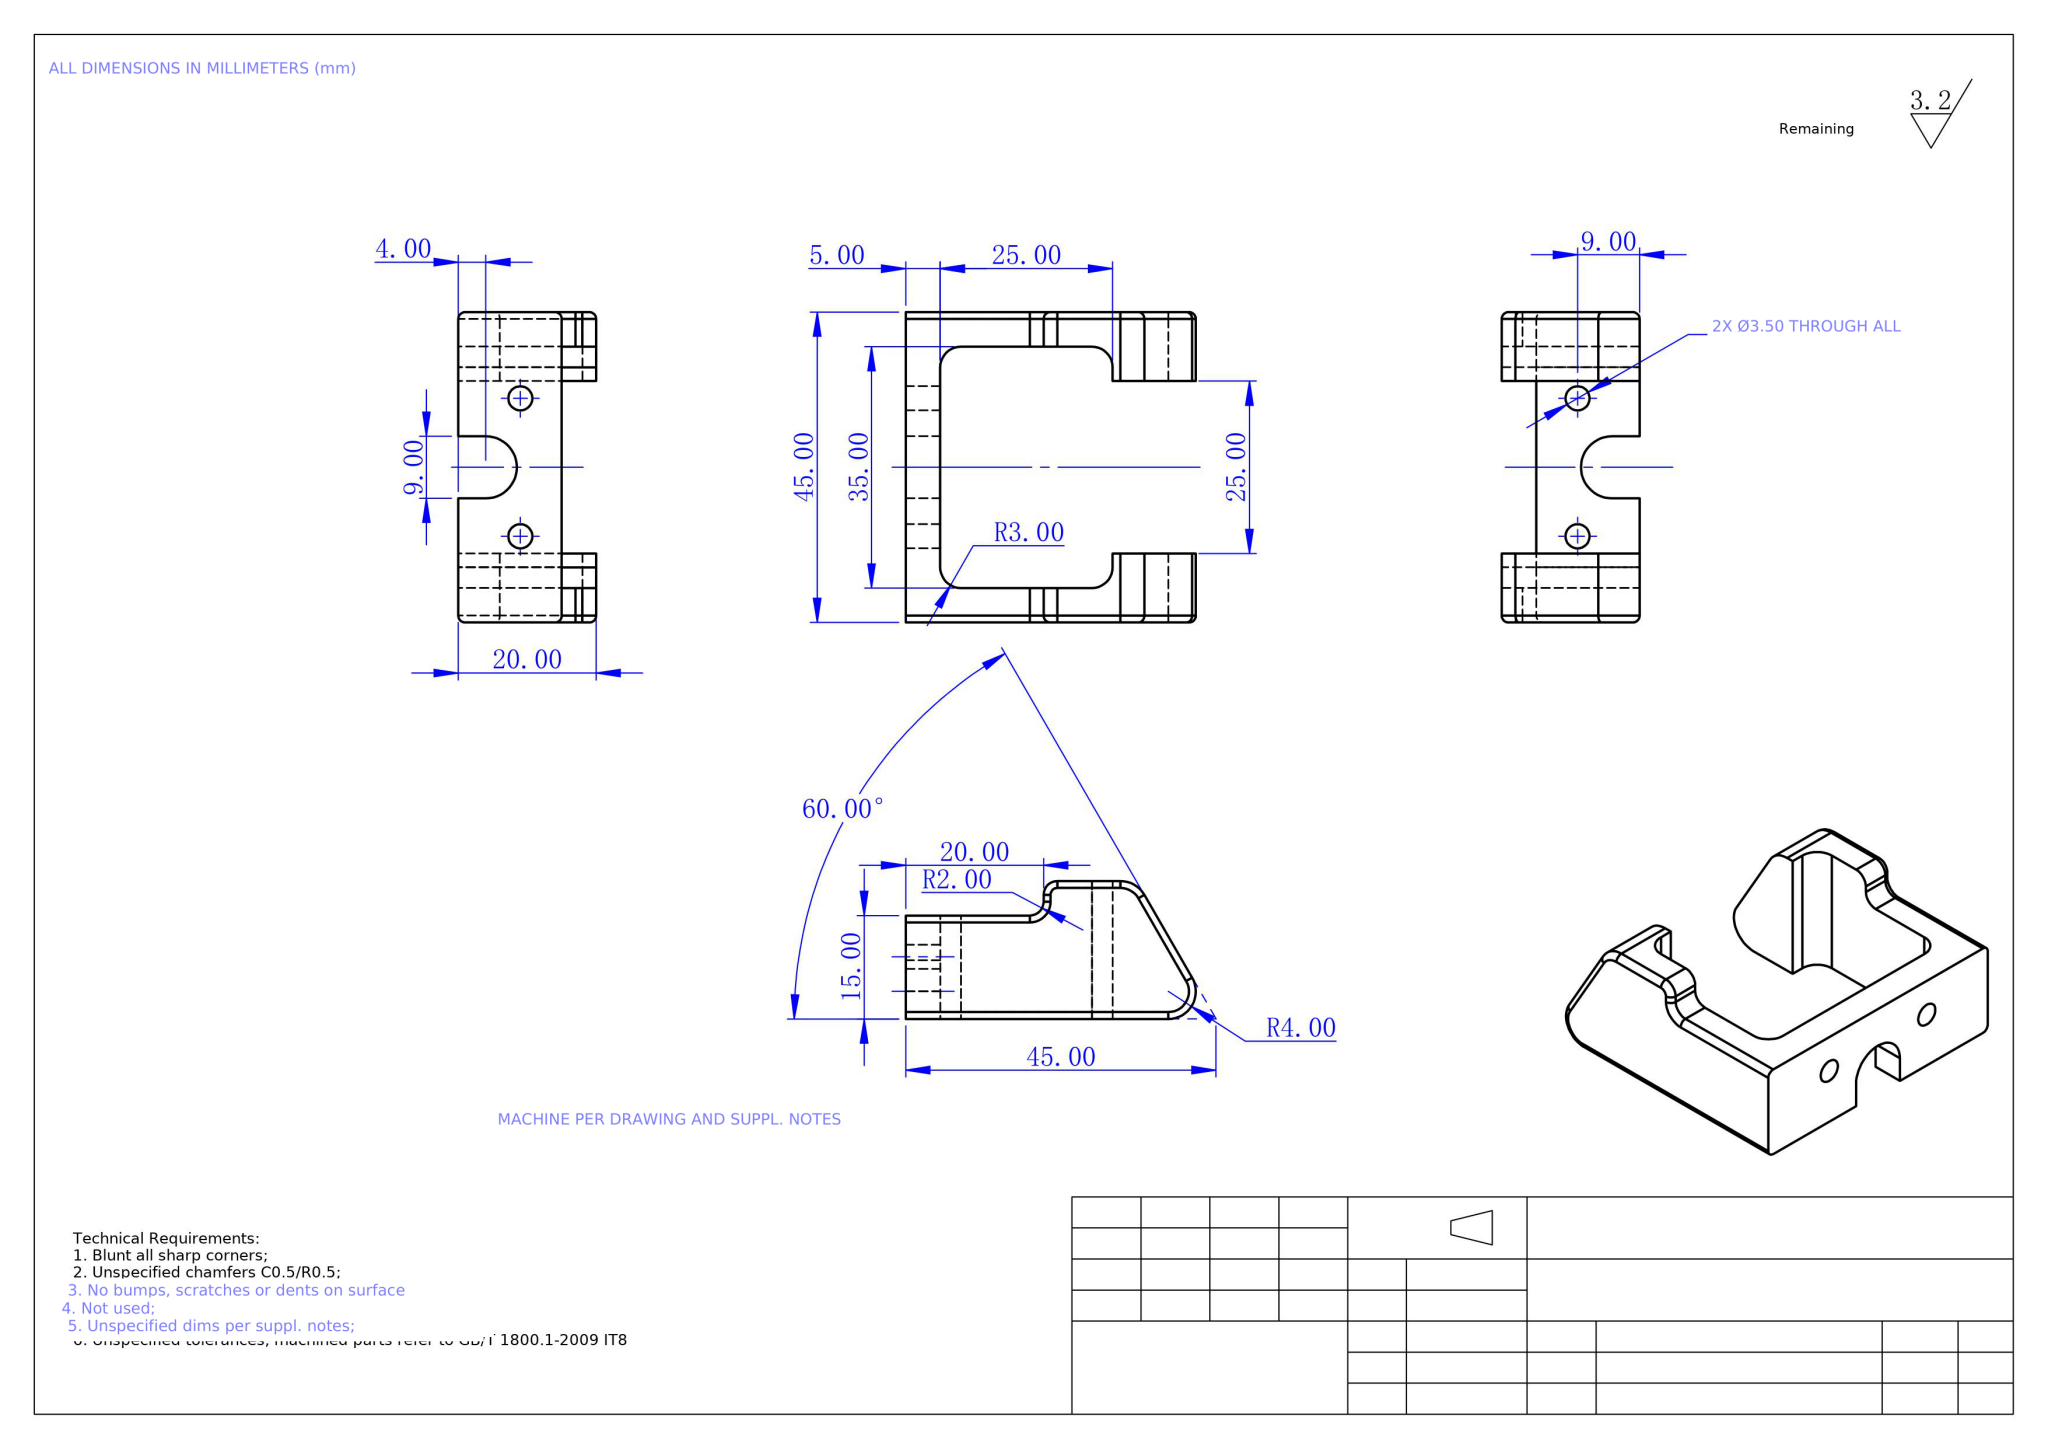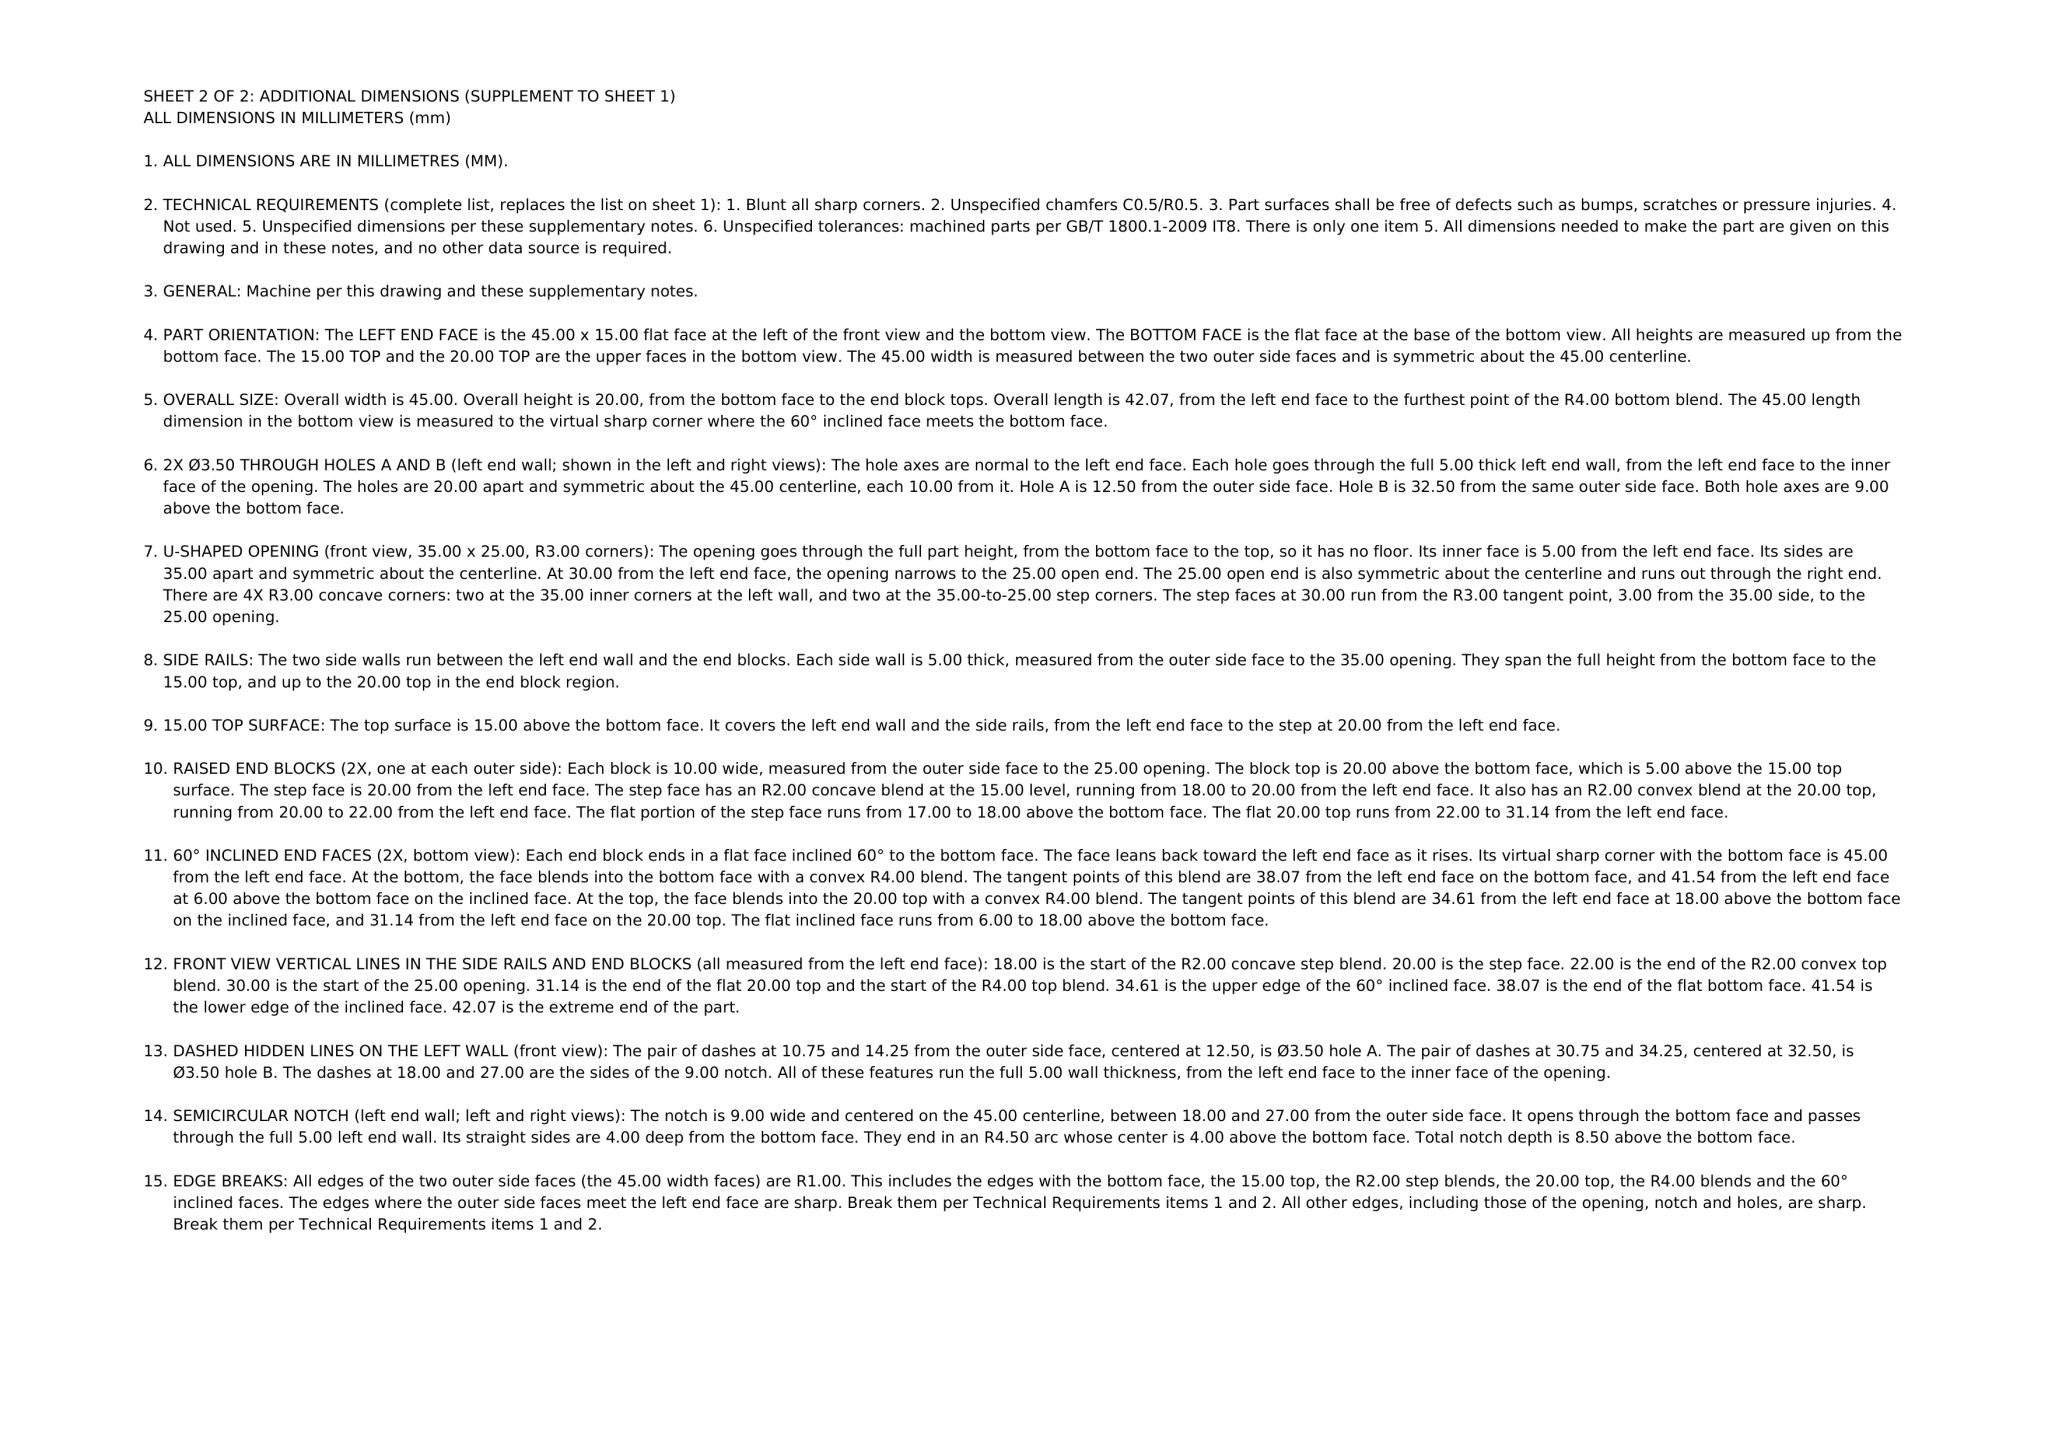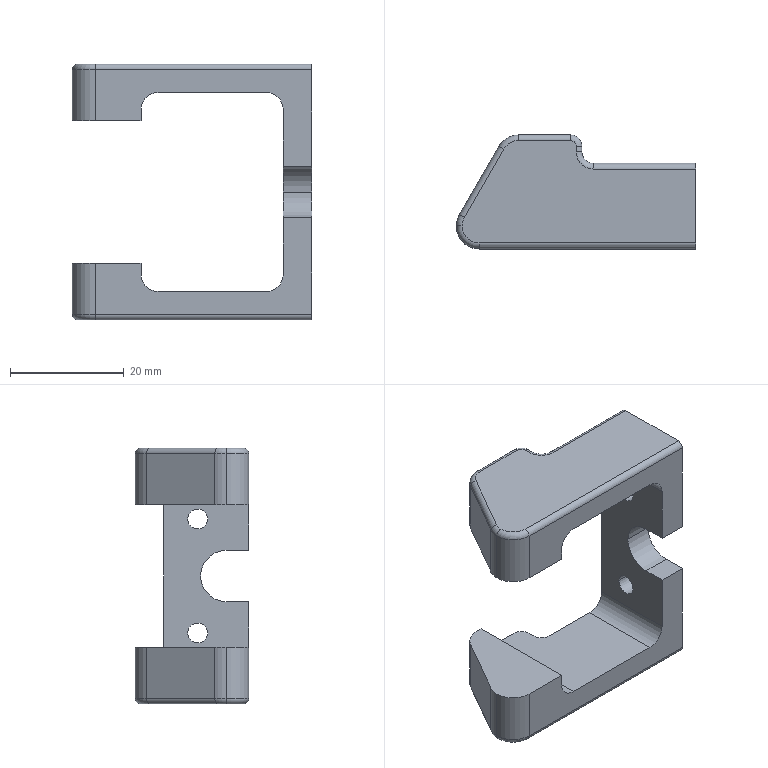Part | NX | mm | 1 solid | 61 faces | box 42.07 x 20 x 45 mm | volume 10737 mm3 | cylinder 30 | plane 21 | torus 10 | commonest cylinder face diameters 2 x10 8 x6 3.5 x4 6 x4 4 x4 9 x2